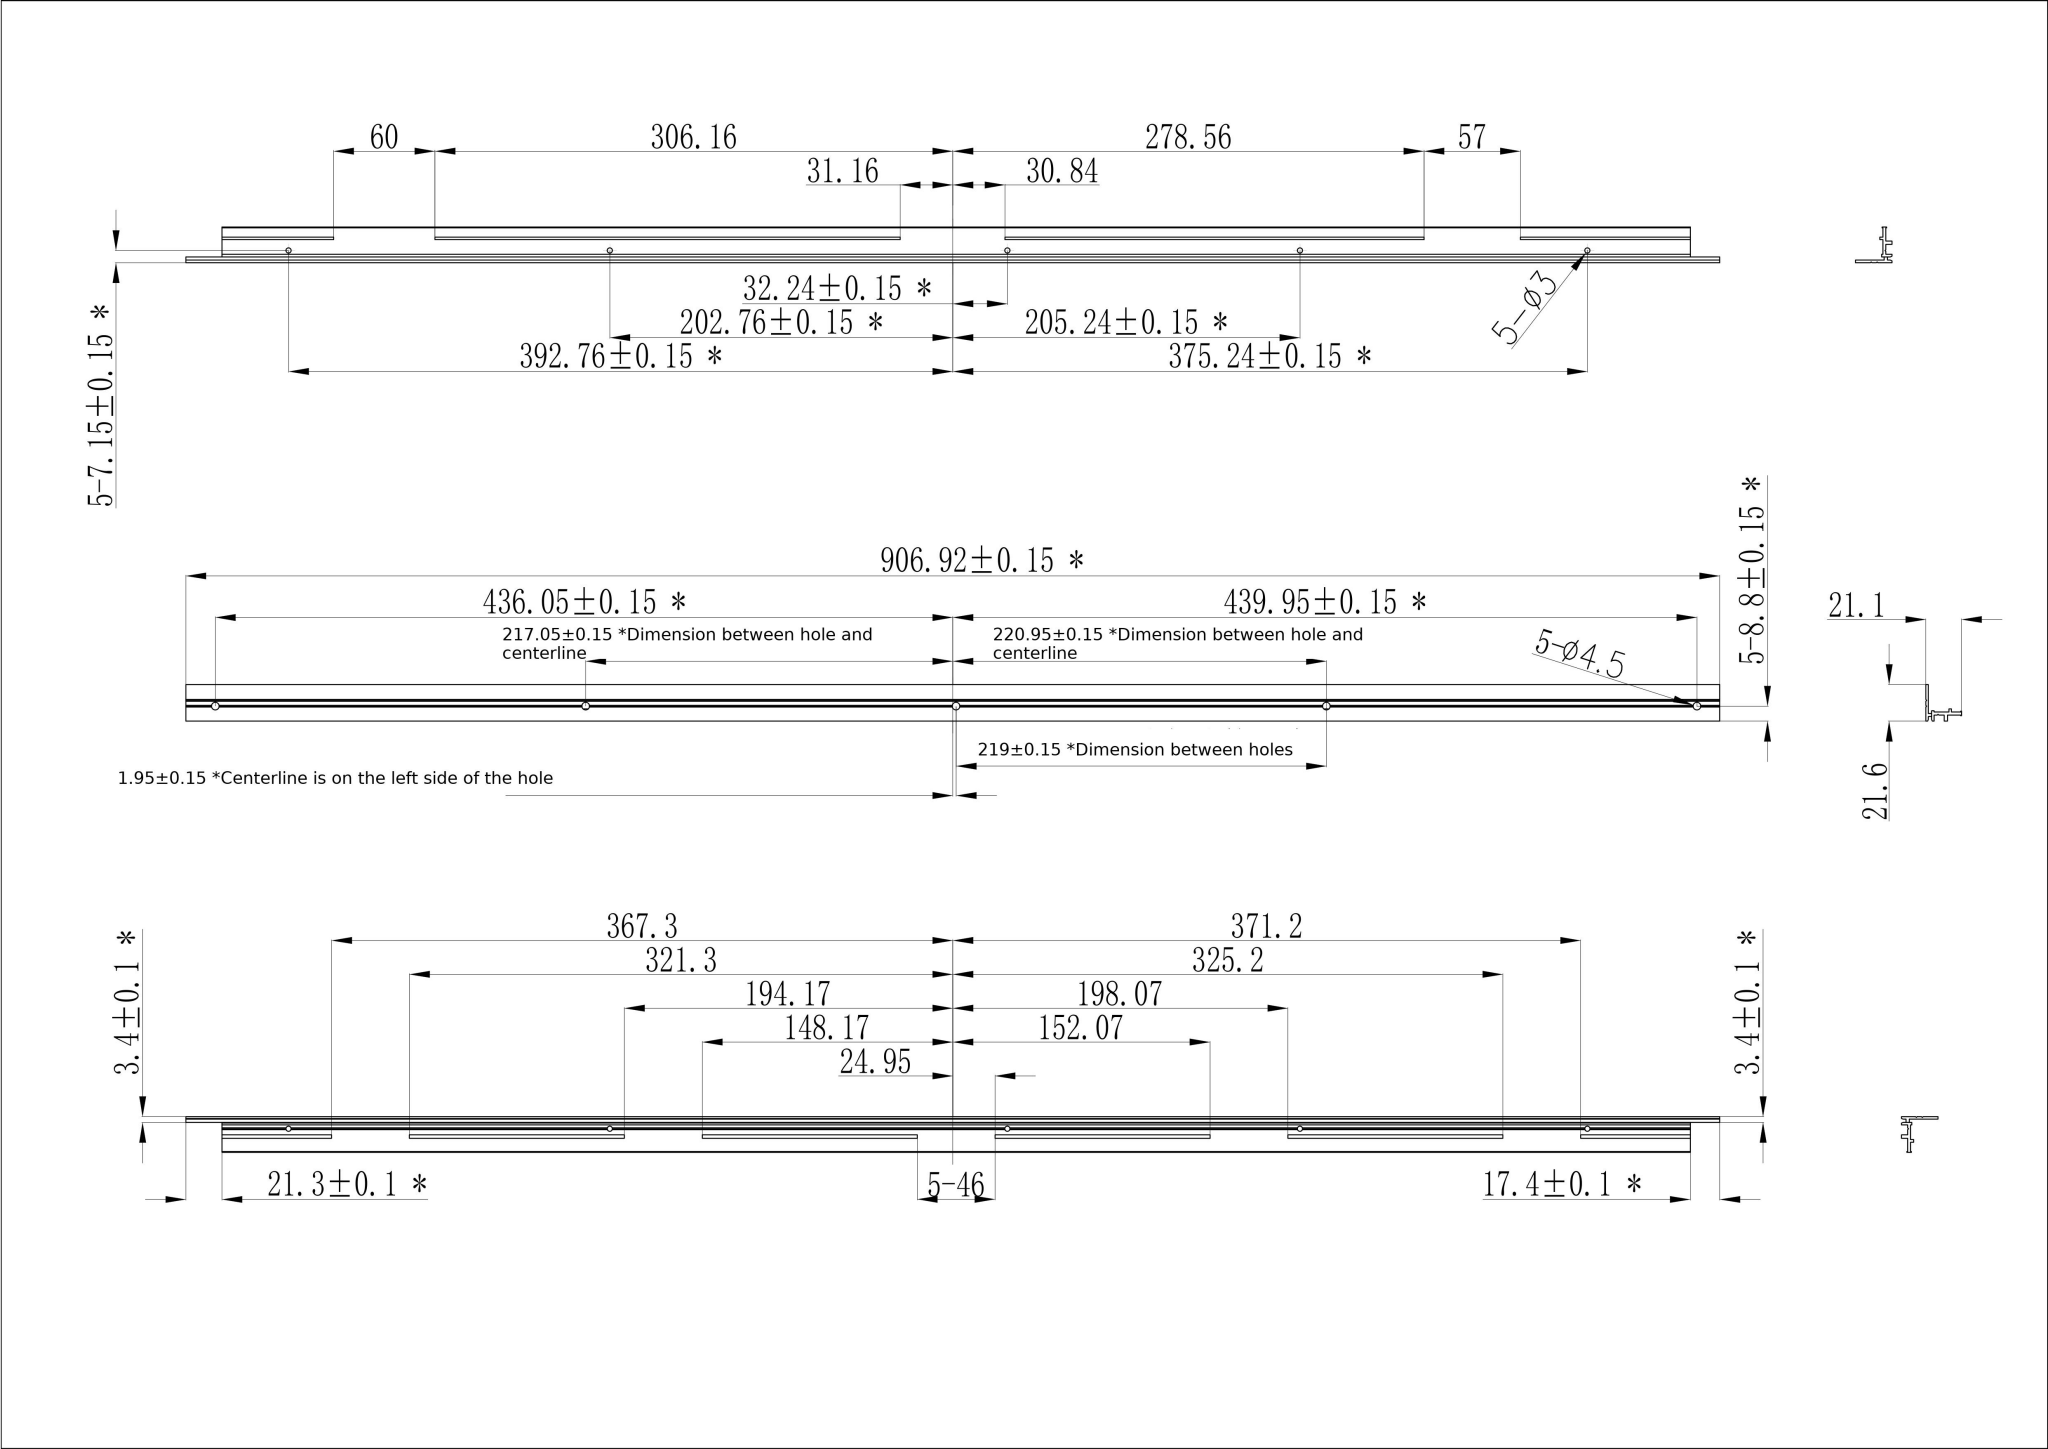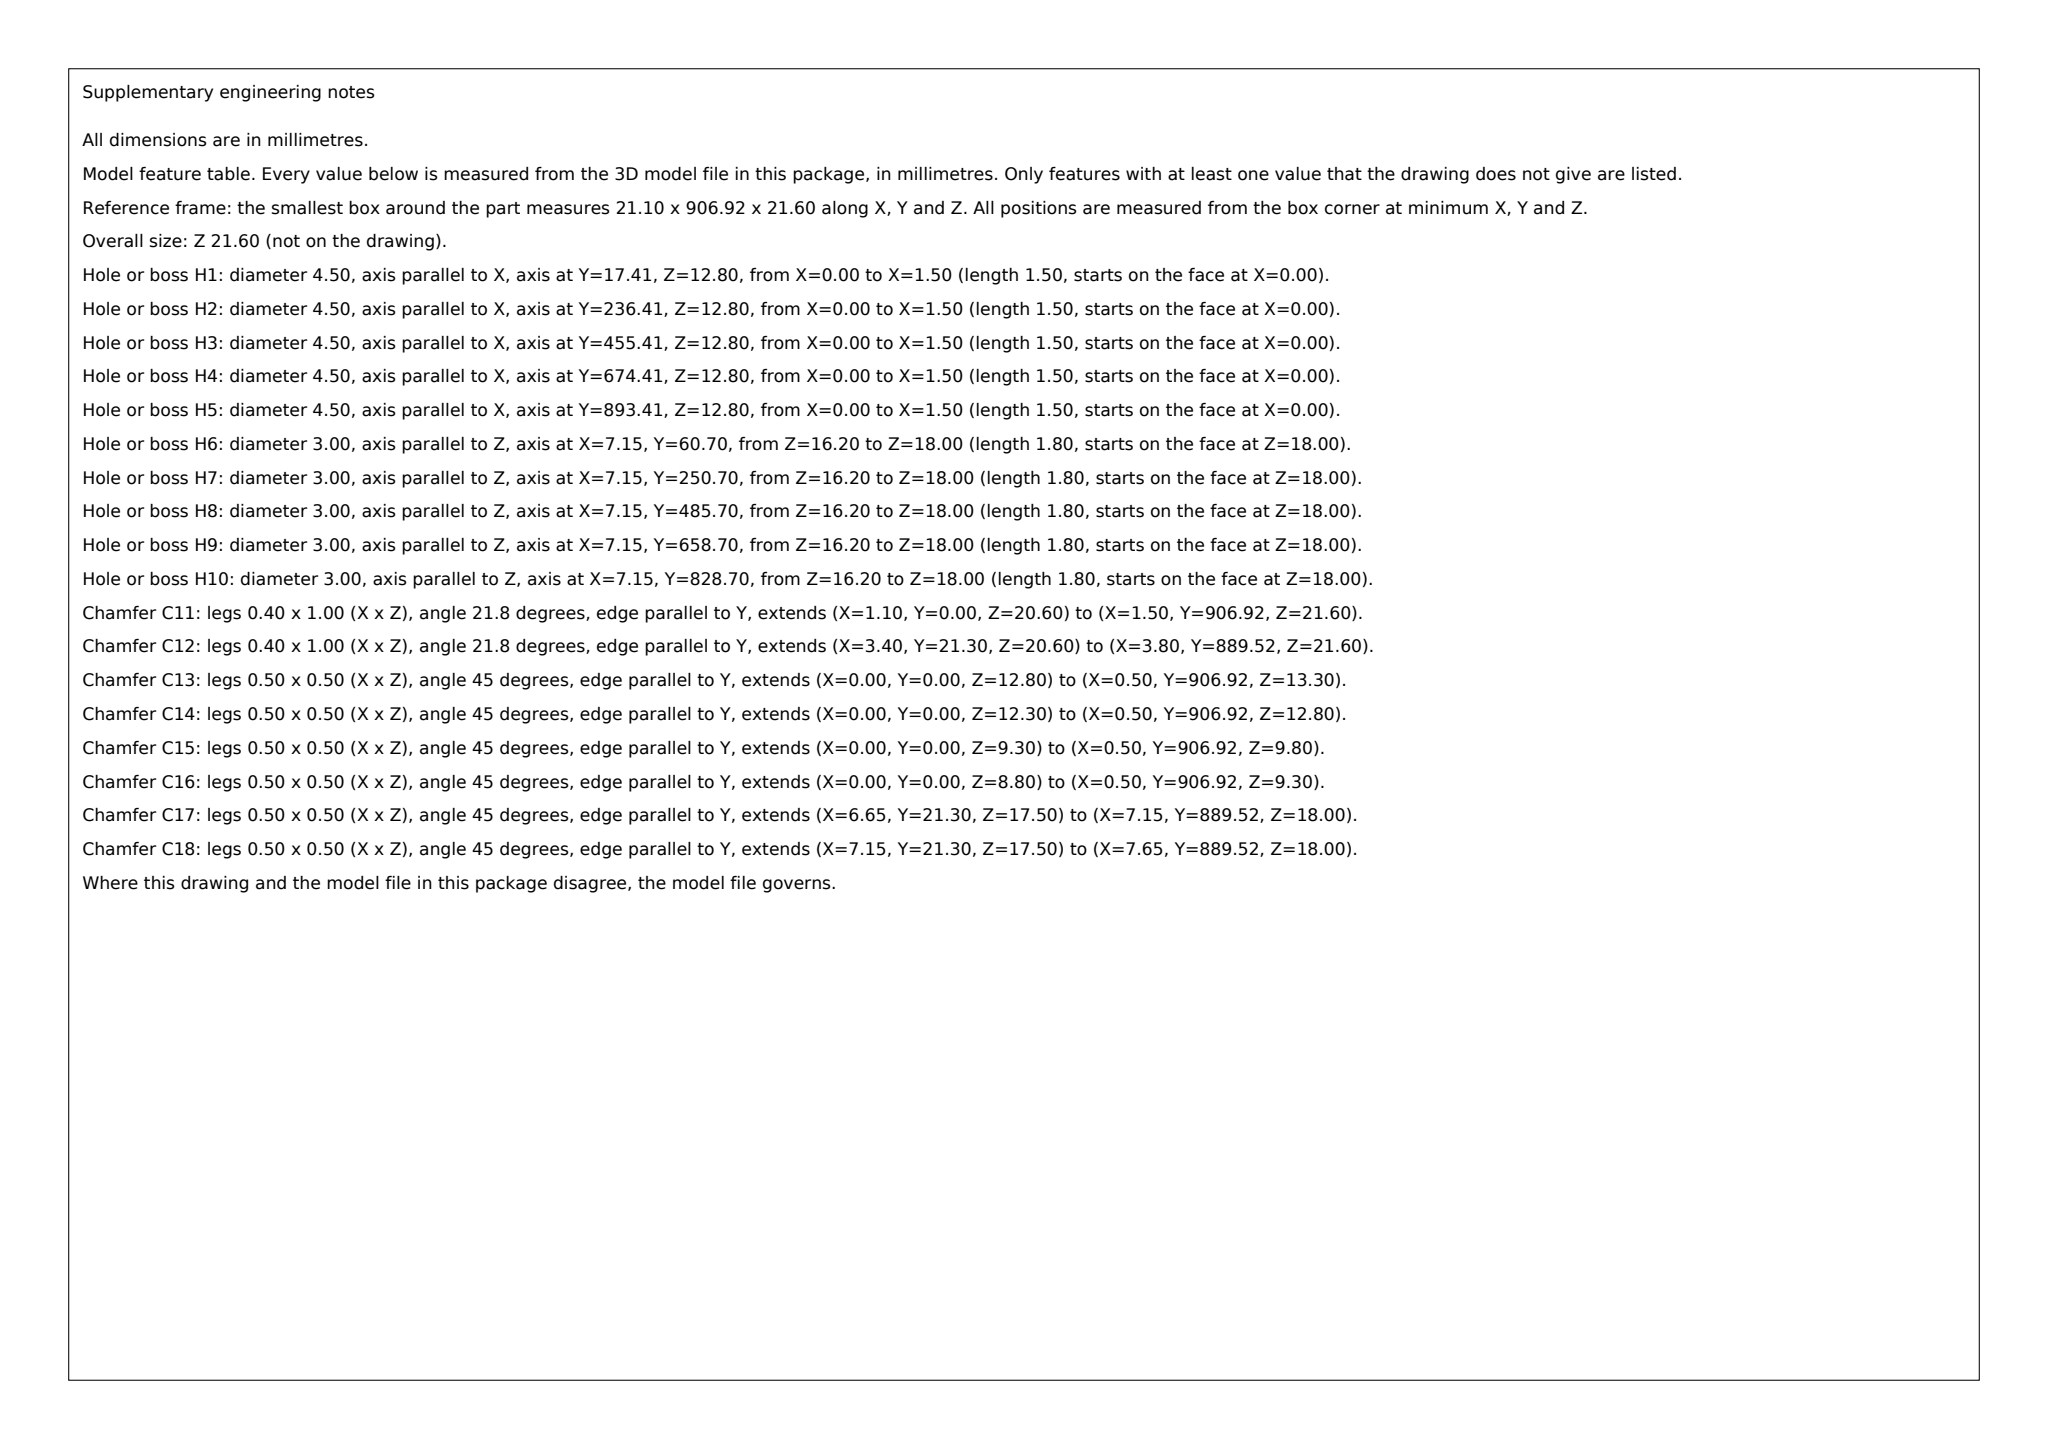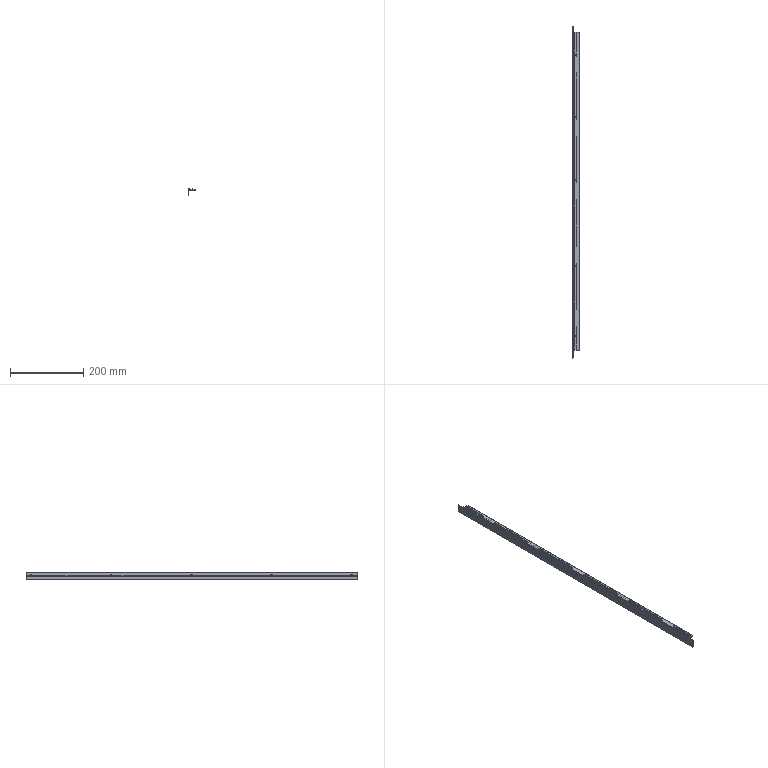Part | SolidWorks | mm | 1 solid | 123 faces | box 21.1 x 906.92 x 21.6 mm | volume 71567 mm3 | plane 103 | cylinder 20 | commonest cylinder face diameters 4.5 x10 3 x10